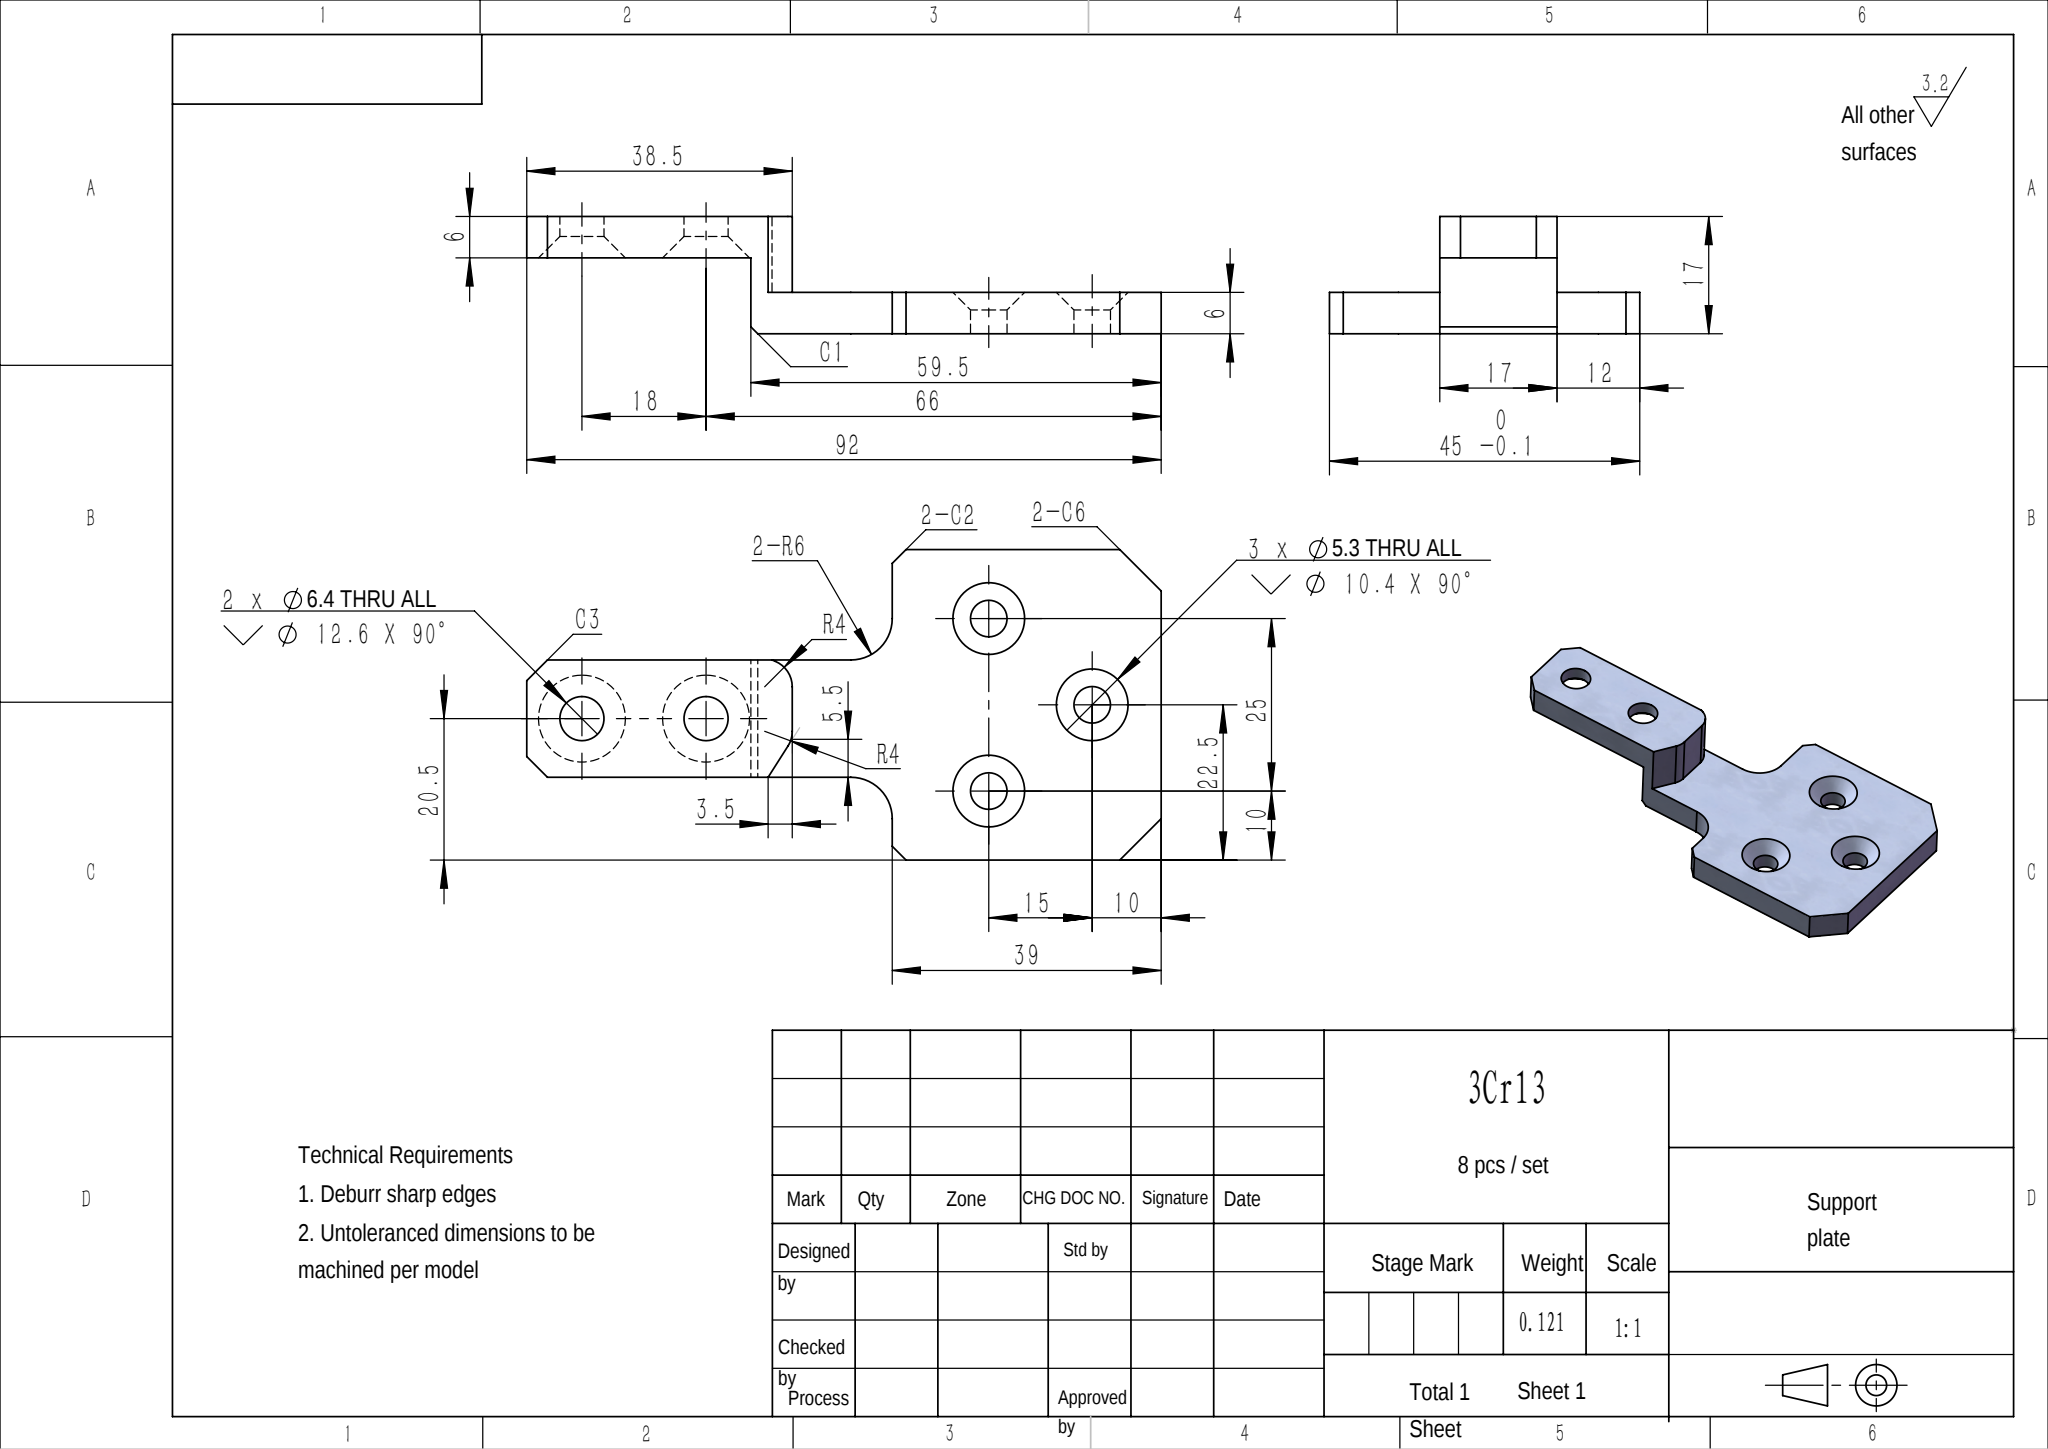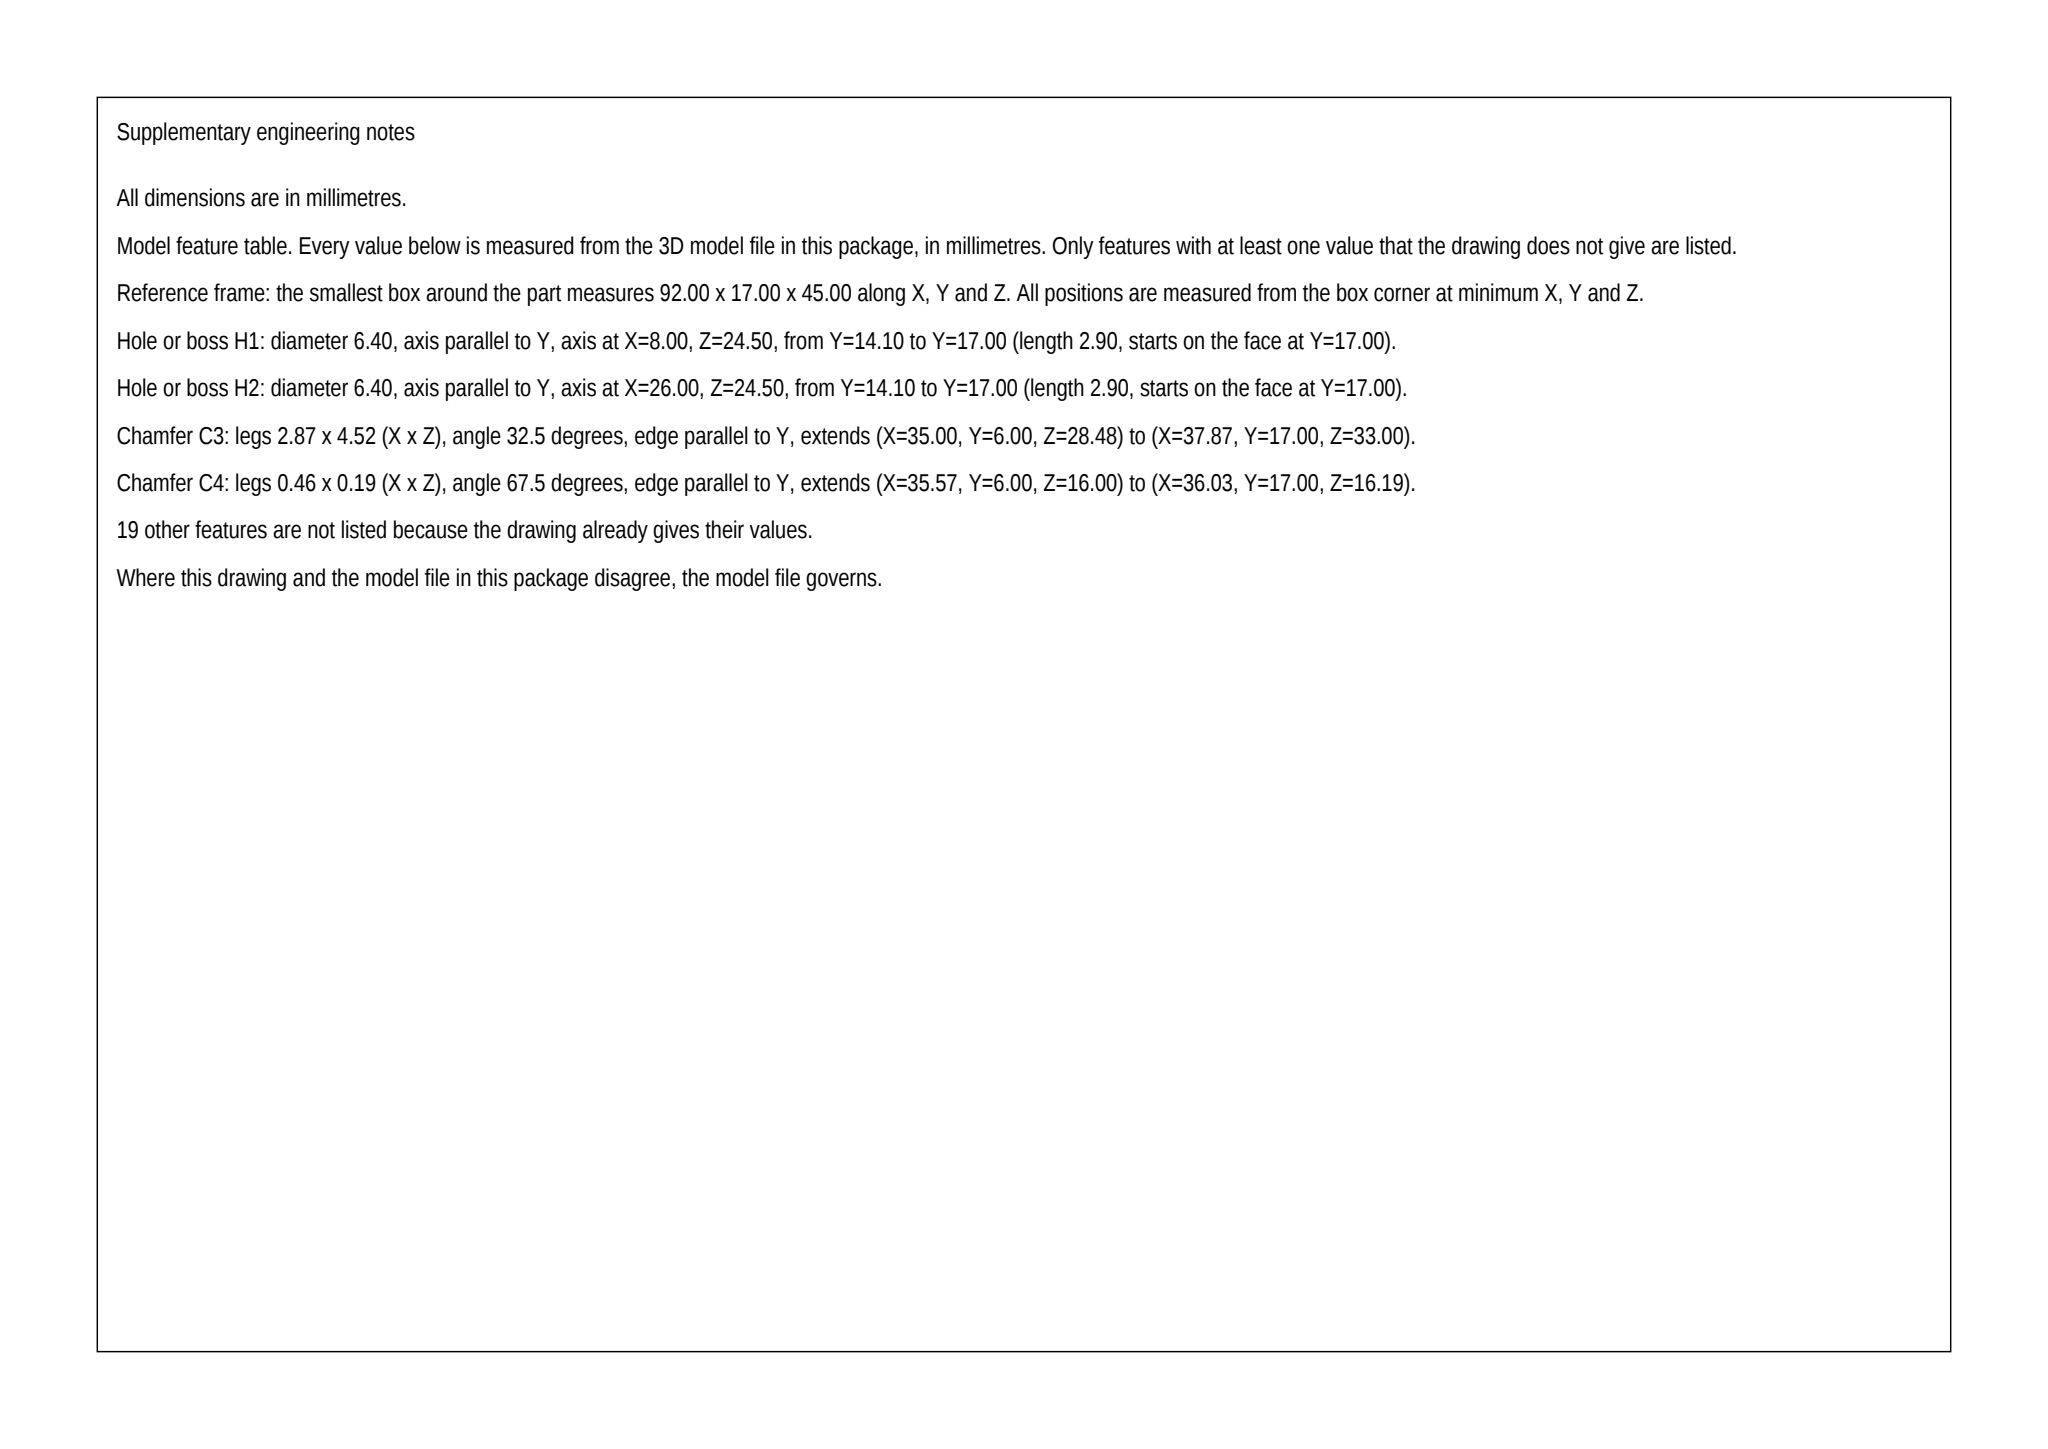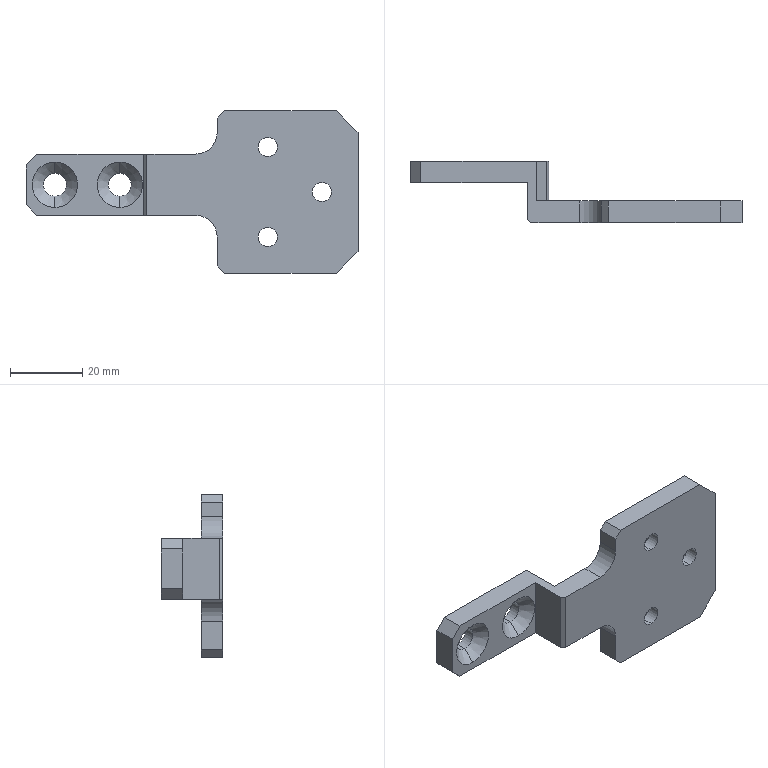Part | SolidWorks | mm | material 3Cr13 | 1 solid | 47 faces | box 92 x 17 x 45 mm | volume 15454 mm3 | plane 23 | cylinder 14 | cone 10 | commonest cylinder face diameters 5.3 x6 6.4 x4 12 x2 8 x2